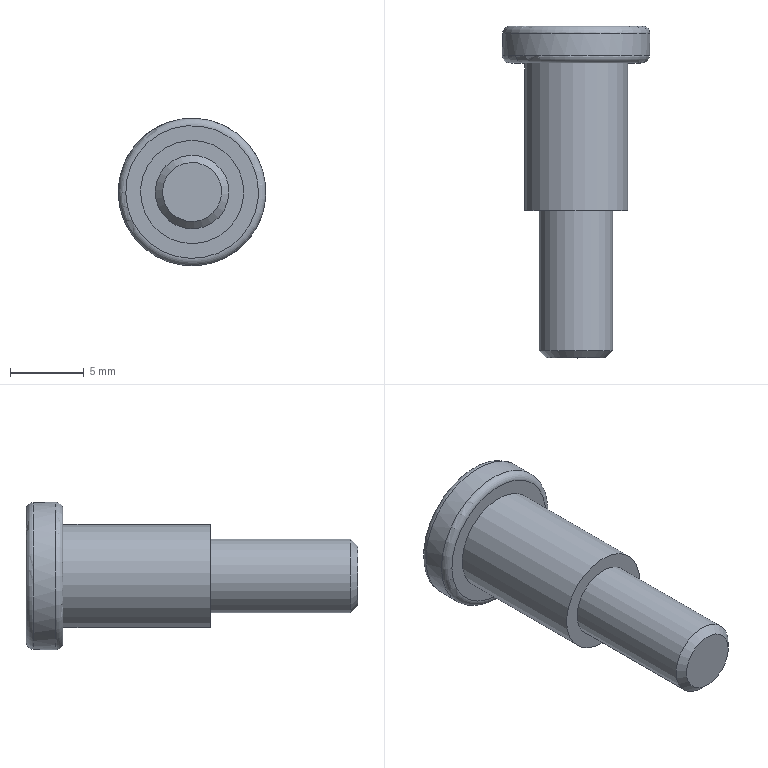Component | NX | CONNECTING_PIN | 1 solid | 10 faces | volume 772 mm3 | plane 4 | cylinder 3 | torus 2 | cone 1 | commonest cylinder face diameters 10 x1 7 x1 5 x1